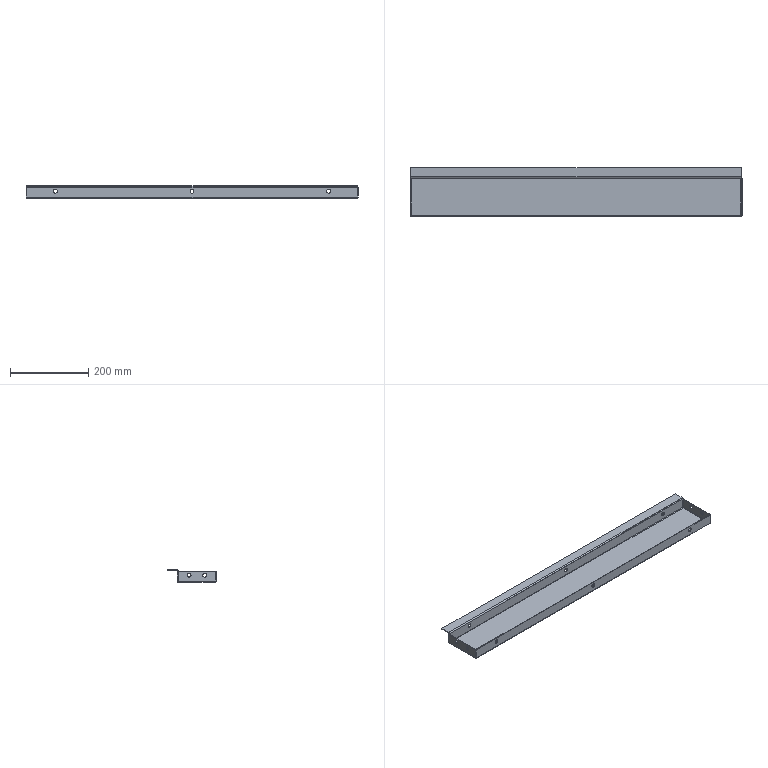Component | SolidWorks | 27BaseRearSidePlateII-1 | 1 solid | 66 faces | volume 310640 mm3 | cylinder 30 | plane 28 | spline 8 | commonest cylinder face diameters 10 x20 2 x5 6 x5